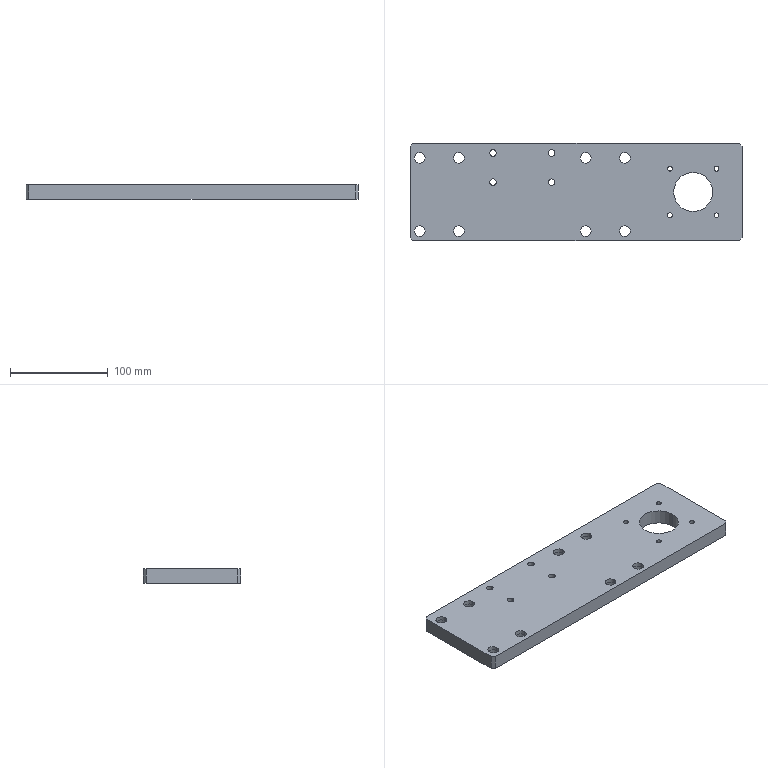Component | SolidWorks | -UpperSlidingSleeveConnectingPlate01-1 | 1 solid | 80 faces | box 340 x 100 x 15 mm | volume 462800 mm3 | cylinder 56 | plane 18 | cone 6 | commonest cylinder face diameters 11 x16 17 x16 6.8 x14 5 x8 40 x2
build123d program:
from build123d import *

# Parameters (mm, degrees)
SKETCH1_W             = 340
SKETCH1_H             = 100
BOSS_EXTRUDE1_DEPTH   = 7.5
LPATTERN1_COUNT       = 2
LPATTERN1_PITCH       = 40
LPATTERN1_COUNT_DIR2  = 2
LPATTERN1_PITCH_DIR2  = 75
LPATTERN2_COUNT       = 2
LPATTERN2_PITCH       = 40
LPATTERN2_COUNT_DIR2  = 2
LPATTERN2_PITCH_DIR2  = 75
SKETCH6_R             = 20
CUT_EXTRUDE1_DEPTH    = 15
CIRPATTERN1_COUNT     = 4
M8_TAPPED_HOLE2_D     = 6.8
M8_TAPPED_HOLE2_DEPTH = 15
M8_TAPPED_HOLE2_TIP   = 2.043
CHAMFER1_SIZE         = 3
M8_TAPPED_HOLE3_D     = 6.8


with BuildPart() as part:
    # Sketch1 → Boss-Extrude1 (new, symmetric)
    with BuildSketch(Plane.XY):
        Rectangle(SKETCH1_W, SKETCH1_H)
    extrude(amount=BOSS_EXTRUDE1_DEPTH, both=True)

    # Sketch2 → Cylindrical Countersunk Hole for M10 Hex (revolve, cut)
    with BuildSketch(Plane(origin=(-120, 35, -7.5), x_dir=(0, 1, 0), z_dir=(1, 0, 0))):
        Polygon((0, 0), (0, 25.555), (5.5, 22.25), (5.5, 11), (8.5, 11), (8.5, 0), align=None)
    cylindrical_countersunk_hole_for_m10_hex = revolve(axis=Axis((-120, 35, -13.85), (0, 0, 1)), mode=Mode.SUBTRACT)

    # LPattern1: Cylindrical Countersunk Hole for M10 Hex 2 × 2
    with Locations(*[(-i * LPATTERN1_PITCH, -j * LPATTERN1_PITCH_DIR2, 0) for i in range(LPATTERN1_COUNT) for j in range(LPATTERN1_COUNT_DIR2) if (i, j) != (0, 0)]):
        add(cylindrical_countersunk_hole_for_m10_hex, mode=Mode.SUBTRACT)

    # Sketch4 → Cylindrical Countersunk Hole for M10 2 (revolve, cut)
    with BuildSketch(Plane(origin=(50, 35, -7.5), x_dir=(0, 1, 0), z_dir=(1, 0, 0))):
        Polygon((0, 0), (0, 25.555), (5.5, 22.25), (5.5, 11), (8.5, 11), (8.5, 0), align=None)
    cylindrical_countersunk_hole_for_m10_2 = revolve(axis=Axis((50, 35, -13.85), (0, 0, 1)), mode=Mode.SUBTRACT)

    # LPattern2: Cylindrical Countersunk Hole for M10 2 2 × 2
    with Locations(*[(-i * LPATTERN2_PITCH, -j * LPATTERN2_PITCH_DIR2, 0) for i in range(LPATTERN2_COUNT) for j in range(LPATTERN2_COUNT_DIR2) if (i, j) != (0, 0)]):
        add(cylindrical_countersunk_hole_for_m10_2, mode=Mode.SUBTRACT)

    # Sketch6 → Cut-Extrude1 (cut)
    with BuildSketch(Plane.XY.offset(7.5)):
        with Locations((120, 0)):
            Circle(SKETCH6_R)
    extrude(amount=-CUT_EXTRUDE1_DEPTH, mode=Mode.SUBTRACT)

    # Sketch7 → M6 Tapped Hole1 (revolve, cut)
    with BuildSketch(Plane(origin=(96.135, 23.865, 7.5), x_dir=(0, -1, 0), z_dir=(1, 0, 0))):
        Polygon((0, 0), (0, 18.502), (2.5, 17), (2.5, 0), align=None)
    m6_tapped_hole1 = revolve(axis=Axis((96.135, 23.865, 13.85), (0, 0, -1)), mode=Mode.SUBTRACT)

    # CirPattern1: M6 Tapped Hole1 ×4 about axis
    cirpattern1_axis = Axis((120, 0, 0), (0, 0, 1))
    for i in range(1, CIRPATTERN1_COUNT):
        add(m6_tapped_hole1.rotate(cirpattern1_axis, i * 360 / CIRPATTERN1_COUNT), mode=Mode.SUBTRACT)

    # M8 Tapped Hole2
    with Locations(Plane(origin=(0, 50, 0), x_dir=(1, 0, 0), z_dir=(0, 1, 0))):
        with Locations((145, 0), (120, 0), (95, 0)):
            Hole(M8_TAPPED_HOLE2_D / 2, depth=M8_TAPPED_HOLE2_DEPTH)
            with Locations((0, 0, -(M8_TAPPED_HOLE2_DEPTH + M8_TAPPED_HOLE2_TIP / 2))):  # 118° drill point
                Cone(0, M8_TAPPED_HOLE2_D / 2, M8_TAPPED_HOLE2_TIP, mode=Mode.SUBTRACT)

    # Chamfer1
    chamfer1_edges = [part.edges().sort_by_distance(p)[0] for p in [
        (170, -50, 0),
        (-170, -50, 0),
        (-170, 50, 0),
        (170, 50, 0),
    ]]
    chamfer(chamfer1_edges, length=CHAMFER1_SIZE)

    # M8 Tapped Hole3 (through all)
    with Locations(Plane(origin=(0, 0, -7.5), x_dir=(-1, 0, 0), z_dir=(0, 0, -1))):
        with Locations((25, 40), (25, 10), (85, 40), (85, 10)):
            Hole(M8_TAPPED_HOLE3_D / 2)


solid = part.part

# Placed as in the assembly
solid = solid.moved(Location((85, 1239.5, -77.5), (0, 0, 0)))